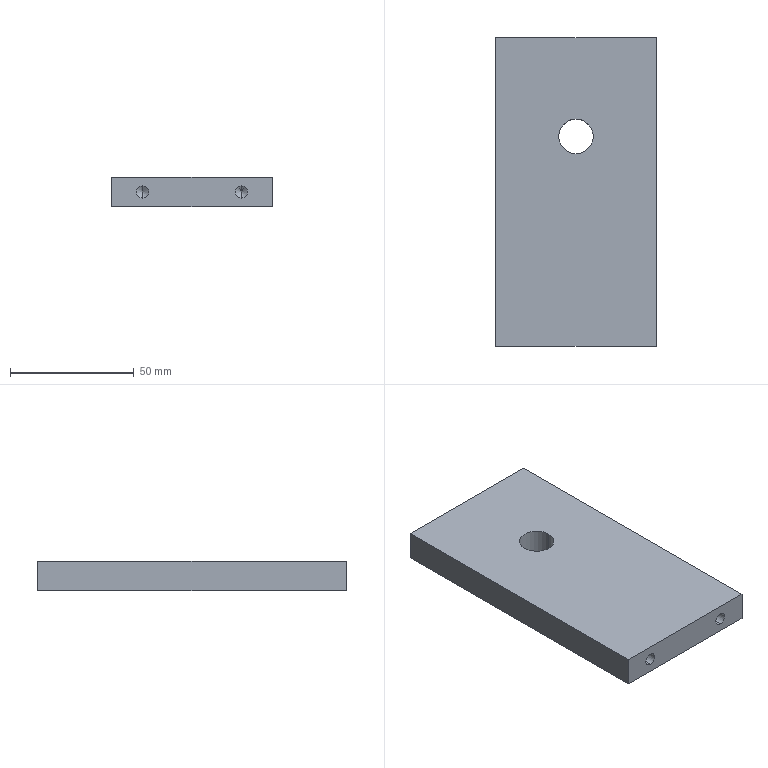Component | SolidWorks | TractionVerticalPlate-1 | 1 solid | 24 faces | box 65 x 125 x 12 mm | volume 94278 mm3 | cylinder 10 | cone 8 | plane 6 | commonest cylinder face diameters 5 x8 14 x2
build123d program:
from build123d import *

# Parameters (mm, degrees)
SKETCH1_W             = 65
SKETCH1_H             = 125
SKETCH1_R             = 7
EXTRUDE1_DEPTH        = 12
M6_TAPPED_HOLE1_D     = 5
M6_TAPPED_HOLE1_DEPTH = 17
M6_TAPPED_HOLE1_TIP   = 1.502
M6_TAPPED_HOLE2_D     = 5
M6_TAPPED_HOLE2_DEPTH = 17
M6_TAPPED_HOLE2_TIP   = 1.502


with BuildPart() as part:
    # Sketch1 → Extrude1 (new body)
    with BuildSketch(Plane.XY):
        Rectangle(SKETCH1_W, SKETCH1_H)
        with Locations((0, 22.5)):
            Circle(SKETCH1_R, mode=Mode.SUBTRACT)
    extrude(amount=EXTRUDE1_DEPTH)

    # M6 Tapped Hole1
    with Locations(Plane(origin=(0, 62.5, 0), x_dir=(-1, 0, 0), z_dir=(0, 1, 0))):
        with Locations((20, 6), (-20, 6)):
            Hole(M6_TAPPED_HOLE1_D / 2, depth=M6_TAPPED_HOLE1_DEPTH)
            with Locations((0, 0, -(M6_TAPPED_HOLE1_DEPTH + M6_TAPPED_HOLE1_TIP / 2))):  # 118° drill point
                Cone(0, M6_TAPPED_HOLE1_D / 2, M6_TAPPED_HOLE1_TIP, mode=Mode.SUBTRACT)

    # M6 Tapped Hole2
    with Locations(Plane.XZ.offset(62.5)):
        with Locations((20, 6), (-20, 6)):
            Hole(M6_TAPPED_HOLE2_D / 2, depth=M6_TAPPED_HOLE2_DEPTH)
            with Locations((0, 0, -(M6_TAPPED_HOLE2_DEPTH + M6_TAPPED_HOLE2_TIP / 2))):  # 118° drill point
                Cone(0, M6_TAPPED_HOLE2_D / 2, M6_TAPPED_HOLE2_TIP, mode=Mode.SUBTRACT)


solid = part.part

# Placed as in the assembly
solid = solid.moved(Location((250.216, 449.483, 260.5), (0, 0, 0)))
STEP:
#1=COLOUR_RGB('',0.7922,0.8196,0.9333);
#2=FILL_AREA_STYLE_COLOUR('',#1);
#3=FILL_AREA_STYLE('',(#2));
#4=SURFACE_STYLE_FILL_AREA(#3);
#5=SURFACE_SIDE_STYLE('',(#4));
#6=SURFACE_STYLE_USAGE(.BOTH.,#5);
#7=PRESENTATION_STYLE_ASSIGNMENT((#6));
#8=CARTESIAN_POINT('',(10.638,15.905,10.591));
#9=VERTEX_POINT('',#8);
#10=CARTESIAN_POINT('',(10.638,15.905,10.394));
#11=VERTEX_POINT('',#10);
#12=CARTESIAN_POINT('',(10.638,15.905,10.492));
#13=DIRECTION('',(0.,-1.,0.));
#14=DIRECTION('',(0.,0.,-1.));
#15=AXIS2_PLACEMENT_3D('',#12,#13,#14);
#16=CIRCLE('',#15,0.09843);
#17=EDGE_CURVE('',#9,#11,#16,.T.);
#18=ORIENTED_EDGE('',*,*,#17,.F.);
#19=CARTESIAN_POINT('',(10.638,15.236,10.591));
#20=VERTEX_POINT('',#19);
#21=CARTESIAN_POINT('',(10.638,15.236,10.591));
#22=DIRECTION('',(0.,-1.,0.));
#23=VECTOR('',#22,39.37);
#24=LINE('',#21,#23);
#25=EDGE_CURVE('',#9,#20,#24,.T.);
#26=ORIENTED_EDGE('',*,*,#25,.T.);
#27=CARTESIAN_POINT('',(10.638,15.236,10.394));
#28=VERTEX_POINT('',#27);
#29=CARTESIAN_POINT('',(10.638,15.236,10.492));
#30=DIRECTION('',(0.,-1.,0.));
#31=DIRECTION('',(0.,0.,-1.));
#32=AXIS2_PLACEMENT_3D('',#29,#30,#31);
#33=CIRCLE('',#32,0.09843);
#34=EDGE_CURVE('',#20,#28,#33,.T.);
#35=ORIENTED_EDGE('',*,*,#34,.T.);
#36=CARTESIAN_POINT('',(10.638,15.236,10.394));
#37=DIRECTION('',(0.,-1.,0.));
#38=VECTOR('',#37,39.37);
#39=LINE('',#36,#38);
#40=EDGE_CURVE('',#11,#28,#39,.T.);
#41=ORIENTED_EDGE('',*,*,#40,.F.);
#42=EDGE_LOOP('',(#18,#26,#35,#41));
#43=FACE_OUTER_BOUND('',#42,.T.);
#44=CARTESIAN_POINT('',(10.638,15.236,10.492));
#45=DIRECTION('',(0.,-1.,0.));
#46=DIRECTION('',(0.,0.,-1.));
#47=AXIS2_PLACEMENT_3D('',#44,#45,#46);
#48=CYLINDRICAL_SURFACE('',#47,0.09843);
#49=ADVANCED_FACE('',(#43),#48,.F.);
#50=CARTESIAN_POINT('',(10.638,15.964,10.492));
#51=VERTEX_POINT('',#50);
#52=CARTESIAN_POINT('',(10.638,15.905,10.394));
#53=DIRECTION('',(0.,-0.515,-0.8572));
#54=VECTOR('',#53,39.37);
#55=LINE('',#52,#54);
#56=EDGE_CURVE('',#51,#11,#55,.T.);
#57=ORIENTED_EDGE('',*,*,#56,.F.);
#58=CARTESIAN_POINT('',(10.638,15.905,10.591));
#59=DIRECTION('',(0.,-0.515,0.8572));
#60=VECTOR('',#59,39.37);
#61=LINE('',#58,#60);
#62=EDGE_CURVE('',#51,#9,#61,.T.);
#63=ORIENTED_EDGE('',*,*,#62,.T.);
#64=ORIENTED_EDGE('',*,*,#17,.T.);
#65=EDGE_LOOP('',(#57,#63,#64));
#66=FACE_OUTER_BOUND('',#65,.T.);
#67=CARTESIAN_POINT('',(10.638,15.905,10.492));
#68=DIRECTION('',(0.,-1.,0.));
#69=DIRECTION('',(0.,0.,-1.));
#70=AXIS2_PLACEMENT_3D('',#67,#68,#69);
#71=CONICAL_SURFACE('',#70,0.09843,1.03);
#72=ADVANCED_FACE('',(#66),#71,.F.);
#73=CARTESIAN_POINT('',(9.064,15.905,10.591));
#74=VERTEX_POINT('',#73);
#75=CARTESIAN_POINT('',(9.064,15.905,10.394));
#76=VERTEX_POINT('',#75);
#77=CARTESIAN_POINT('',(9.064,15.905,10.492));
#78=DIRECTION('',(0.,-1.,0.));
#79=DIRECTION('',(0.,0.,-1.));
#80=AXIS2_PLACEMENT_3D('',#77,#78,#79);
#81=CIRCLE('',#80,0.09843);
#82=EDGE_CURVE('',#74,#76,#81,.T.);
#83=ORIENTED_EDGE('',*,*,#82,.F.);
#84=CARTESIAN_POINT('',(9.064,15.236,10.591));
#85=VERTEX_POINT('',#84);
#86=CARTESIAN_POINT('',(9.064,15.236,10.591));
#87=DIRECTION('',(0.,-1.,0.));
#88=VECTOR('',#87,39.37);
#89=LINE('',#86,#88);
#90=EDGE_CURVE('',#74,#85,#89,.T.);
#91=ORIENTED_EDGE('',*,*,#90,.T.);
#92=CARTESIAN_POINT('',(9.064,15.236,10.394));
#93=VERTEX_POINT('',#92);
#94=CARTESIAN_POINT('',(9.064,15.236,10.492));
#95=DIRECTION('',(0.,-1.,0.));
#96=DIRECTION('',(0.,0.,-1.));
#97=AXIS2_PLACEMENT_3D('',#94,#95,#96);
#98=CIRCLE('',#97,0.09843);
#99=EDGE_CURVE('',#85,#93,#98,.T.);
#100=ORIENTED_EDGE('',*,*,#99,.T.);
#101=CARTESIAN_POINT('',(9.064,15.236,10.394));
#102=DIRECTION('',(0.,-1.,0.));
#103=VECTOR('',#102,39.37);
#104=LINE('',#101,#103);
#105=EDGE_CURVE('',#76,#93,#104,.T.);
#106=ORIENTED_EDGE('',*,*,#105,.F.);
#107=EDGE_LOOP('',(#83,#91,#100,#106));
#108=FACE_OUTER_BOUND('',#107,.T.);
#109=CARTESIAN_POINT('',(9.064,15.236,10.492));
#110=DIRECTION('',(0.,-1.,0.));
#111=DIRECTION('',(0.,0.,-1.));
#112=AXIS2_PLACEMENT_3D('',#109,#110,#111);
#113=CYLINDRICAL_SURFACE('',#112,0.09843);
#114=ADVANCED_FACE('',(#108),#113,.F.);
#115=CARTESIAN_POINT('',(9.064,15.964,10.492));
#116=VERTEX_POINT('',#115);
#117=CARTESIAN_POINT('',(9.064,15.905,10.394));
#118=DIRECTION('',(0.,-0.515,-0.8572));
#119=VECTOR('',#118,39.37);
#120=LINE('',#117,#119);
#121=EDGE_CURVE('',#116,#76,#120,.T.);
#122=ORIENTED_EDGE('',*,*,#121,.F.);
#123=CARTESIAN_POINT('',(9.064,15.905,10.591));
#124=DIRECTION('',(0.,-0.515,0.8572));
#125=VECTOR('',#124,39.37);
#126=LINE('',#123,#125);
#127=EDGE_CURVE('',#116,#74,#126,.T.);
#128=ORIENTED_EDGE('',*,*,#127,.T.);
#129=ORIENTED_EDGE('',*,*,#82,.T.);
#130=EDGE_LOOP('',(#122,#128,#129));
#131=FACE_OUTER_BOUND('',#130,.T.);
#132=CARTESIAN_POINT('',(9.064,15.905,10.492));
#133=DIRECTION('',(0.,-1.,0.));
#134=DIRECTION('',(0.,0.,-1.));
#135=AXIS2_PLACEMENT_3D('',#132,#133,#134);
#136=CONICAL_SURFACE('',#135,0.09843,1.03);
#137=ADVANCED_FACE('',(#131),#136,.F.);
#138=CARTESIAN_POINT('',(9.064,19.488,10.394));
#139=VERTEX_POINT('',#138);
#140=CARTESIAN_POINT('',(9.064,19.488,10.591));
#141=VERTEX_POINT('',#140);
#142=CARTESIAN_POINT('',(9.064,19.488,10.492));
#143=DIRECTION('',(0.,1.,0.));
#144=DIRECTION('',(0.,0.,1.));
#145=AXIS2_PLACEMENT_3D('',#142,#143,#144);
#146=CIRCLE('',#145,0.09843);
#147=EDGE_CURVE('',#139,#141,#146,.T.);
#148=ORIENTED_EDGE('',*,*,#147,.F.);
#149=CARTESIAN_POINT('',(9.064,20.157,10.394));
#150=VERTEX_POINT('',#149);
#151=CARTESIAN_POINT('',(9.064,20.157,10.394));
#152=DIRECTION('',(0.,1.,0.));
#153=VECTOR('',#152,39.37);
#154=LINE('',#151,#153);
#155=EDGE_CURVE('',#139,#150,#154,.T.);
#156=ORIENTED_EDGE('',*,*,#155,.T.);
#157=CARTESIAN_POINT('',(9.064,20.157,10.591));
#158=VERTEX_POINT('',#157);
#159=CARTESIAN_POINT('',(9.064,20.157,10.492));
#160=DIRECTION('',(0.,1.,0.));
#161=DIRECTION('',(0.,0.,1.));
#162=AXIS2_PLACEMENT_3D('',#159,#160,#161);
#163=CIRCLE('',#162,0.09843);
#164=EDGE_CURVE('',#150,#158,#163,.T.);
#165=ORIENTED_EDGE('',*,*,#164,.T.);
#166=CARTESIAN_POINT('',(9.064,20.157,10.591));
#167=DIRECTION('',(0.,1.,0.));
#168=VECTOR('',#167,39.37);
#169=LINE('',#166,#168);
#170=EDGE_CURVE('',#141,#158,#169,.T.);
#171=ORIENTED_EDGE('',*,*,#170,.F.);
#172=EDGE_LOOP('',(#148,#156,#165,#171));
#173=FACE_OUTER_BOUND('',#172,.T.);
#174=CARTESIAN_POINT('',(9.064,20.157,10.492));
#175=DIRECTION('',(0.,1.,0.));
#176=DIRECTION('',(0.,0.,1.));
#177=AXIS2_PLACEMENT_3D('',#174,#175,#176);
#178=CYLINDRICAL_SURFACE('',#177,0.09843);
#179=ADVANCED_FACE('',(#173),#178,.F.);
#180=CARTESIAN_POINT('',(9.064,19.428,10.492));
#181=VERTEX_POINT('',#180);
#182=CARTESIAN_POINT('',(9.064,19.488,10.591));
#183=DIRECTION('',(0.,0.515,0.8572));
#184=VECTOR('',#183,39.37);
#185=LINE('',#182,#184);
#186=EDGE_CURVE('',#181,#141,#185,.T.);
#187=ORIENTED_EDGE('',*,*,#186,.F.);
#188=CARTESIAN_POINT('',(9.064,19.488,10.394));
#189=DIRECTION('',(0.,0.515,-0.8572));
#190=VECTOR('',#189,39.37);
#191=LINE('',#188,#190);
#192=EDGE_CURVE('',#181,#139,#191,.T.);
#193=ORIENTED_EDGE('',*,*,#192,.T.);
#194=ORIENTED_EDGE('',*,*,#147,.T.);
#195=EDGE_LOOP('',(#187,#193,#194));
#196=FACE_OUTER_BOUND('',#195,.T.);
#197=CARTESIAN_POINT('',(9.064,19.488,10.492));
#198=DIRECTION('',(0.,1.,0.));
#199=DIRECTION('',(0.,0.,1.));
#200=AXIS2_PLACEMENT_3D('',#197,#198,#199);
#201=CONICAL_SURFACE('',#200,0.09843,1.03);
#202=ADVANCED_FACE('',(#196),#201,.F.);
#203=CARTESIAN_POINT('',(10.638,19.488,10.394));
#204=VERTEX_POINT('',#203);
#205=CARTESIAN_POINT('',(10.638,19.488,10.591));
#206=VERTEX_POINT('',#205);
#207=CARTESIAN_POINT('',(10.638,19.488,10.492));
#208=DIRECTION('',(0.,1.,0.));
#209=DIRECTION('',(0.,0.,1.));
#210=AXIS2_PLACEMENT_3D('',#207,#208,#209);
#211=CIRCLE('',#210,0.09843);
#212=EDGE_CURVE('',#204,#206,#211,.T.);
#213=ORIENTED_EDGE('',*,*,#212,.F.);
#214=CARTESIAN_POINT('',(10.638,20.157,10.394));
#215=VERTEX_POINT('',#214);
#216=CARTESIAN_POINT('',(10.638,20.157,10.394));
#217=DIRECTION('',(0.,1.,0.));
#218=VECTOR('',#217,39.37);
#219=LINE('',#216,#218);
#220=EDGE_CURVE('',#204,#215,#219,.T.);
#221=ORIENTED_EDGE('',*,*,#220,.T.);
#222=CARTESIAN_POINT('',(10.638,20.157,10.591));
#223=VERTEX_POINT('',#222);
#224=CARTESIAN_POINT('',(10.638,20.157,10.492));
#225=DIRECTION('',(0.,1.,0.));
#226=DIRECTION('',(0.,0.,1.));
#227=AXIS2_PLACEMENT_3D('',#224,#225,#226);
#228=CIRCLE('',#227,0.09843);
#229=EDGE_CURVE('',#215,#223,#228,.T.);
#230=ORIENTED_EDGE('',*,*,#229,.T.);
#231=CARTESIAN_POINT('',(10.638,20.157,10.591));
#232=DIRECTION('',(0.,1.,0.));
#233=VECTOR('',#232,39.37);
#234=LINE('',#231,#233);
#235=EDGE_CURVE('',#206,#223,#234,.T.);
#236=ORIENTED_EDGE('',*,*,#235,.F.);
#237=EDGE_LOOP('',(#213,#221,#230,#236));
#238=FACE_OUTER_BOUND('',#237,.T.);
#239=CARTESIAN_POINT('',(10.638,20.157,10.492));
#240=DIRECTION('',(0.,1.,0.));
#241=DIRECTION('',(0.,0.,1.));
#242=AXIS2_PLACEMENT_3D('',#239,#240,#241);
#243=CYLINDRICAL_SURFACE('',#242,0.09843);
#244=ADVANCED_FACE('',(#238),#243,.F.);
#245=CARTESIAN_POINT('',(10.638,19.428,10.492));
#246=VERTEX_POINT('',#245);
#247=CARTESIAN_POINT('',(10.638,19.488,10.591));
#248=DIRECTION('',(0.,0.515,0.8572));
#249=VECTOR('',#248,39.37);
#250=LINE('',#247,#249);
#251=EDGE_CURVE('',#246,#206,#250,.T.);
#252=ORIENTED_EDGE('',*,*,#251,.F.);
#253=CARTESIAN_POINT('',(10.638,19.488,10.394));
#254=DIRECTION('',(0.,0.515,-0.8572));
#255=VECTOR('',#254,39.37);
#256=LINE('',#253,#255);
#257=EDGE_CURVE('',#246,#204,#256,.T.);
#258=ORIENTED_EDGE('',*,*,#257,.T.);
#259=ORIENTED_EDGE('',*,*,#212,.T.);
#260=EDGE_LOOP('',(#252,#258,#259));
#261=FACE_OUTER_BOUND('',#260,.T.);
#262=CARTESIAN_POINT('',(10.638,19.488,10.492));
#263=DIRECTION('',(0.,1.,0.));
#264=DIRECTION('',(0.,0.,1.));
#265=AXIS2_PLACEMENT_3D('',#262,#263,#264);
#266=CONICAL_SURFACE('',#265,0.09843,1.03);
#267=ADVANCED_FACE('',(#261),#266,.F.);
#268=CARTESIAN_POINT('',(9.575,18.582,10.728));
#269=VERTEX_POINT('',#268);
#270=CARTESIAN_POINT('',(10.127,18.582,10.728));
#271=VERTEX_POINT('',#270);
#272=CARTESIAN_POINT('',(9.851,18.582,10.728));
#273=DIRECTION('',(0.,0.,1.));
#274=DIRECTION('',(1.,0.,0.));
#275=AXIS2_PLACEMENT_3D('',#272,#273,#274);
#276=CIRCLE('',#275,0.2756);
#277=EDGE_CURVE('',#269,#271,#276,.T.);
#278=ORIENTED_EDGE('',*,*,#277,.T.);
#279=CARTESIAN_POINT('',(10.127,18.582,10.256));
#280=VERTEX_POINT('',#279);
#281=CARTESIAN_POINT('',(10.127,18.582,10.728));
#282=DIRECTION('',(0.,0.,-1.));
#283=VECTOR('',#282,39.37);
#284=LINE('',#281,#283);
#285=EDGE_CURVE('',#271,#280,#284,.T.);
#286=ORIENTED_EDGE('',*,*,#285,.T.);
#287=CARTESIAN_POINT('',(9.575,18.582,10.256));
#288=VERTEX_POINT('',#287);
#289=CARTESIAN_POINT('',(9.851,18.582,10.256));
#290=DIRECTION('',(0.,0.,1.));
#291=DIRECTION('',(1.,0.,0.));
#292=AXIS2_PLACEMENT_3D('',#289,#290,#291);
#293=CIRCLE('',#292,0.2756);
#294=EDGE_CURVE('',#288,#280,#293,.T.);
#295=ORIENTED_EDGE('',*,*,#294,.F.);
#296=CARTESIAN_POINT('',(9.575,18.582,10.728));
#297=DIRECTION('',(0.,0.,-1.));
#298=VECTOR('',#297,39.37);
#299=LINE('',#296,#298);
#300=EDGE_CURVE('',#269,#288,#299,.T.);
#301=ORIENTED_EDGE('',*,*,#300,.F.);
#302=EDGE_LOOP('',(#278,#286,#295,#301));
#303=FACE_OUTER_BOUND('',#302,.T.);
#304=CARTESIAN_POINT('',(9.851,18.582,10.728));
#305=DIRECTION('',(0.,0.,-1.));
#306=DIRECTION('',(-1.,0.,0.));
#307=AXIS2_PLACEMENT_3D('',#304,#305,#306);
#308=CYLINDRICAL_SURFACE('',#307,0.2756);
#309=ADVANCED_FACE('',(#303),#308,.F.);
#310=CARTESIAN_POINT('',(8.572,20.157,10.728));
#311=VERTEX_POINT('',#310);
#312=CARTESIAN_POINT('',(8.572,15.236,10.728));
#313=VERTEX_POINT('',#312);
#314=CARTESIAN_POINT('',(8.572,20.157,10.728));
#315=DIRECTION('',(0.,-1.,0.));
#316=VECTOR('',#315,39.37);
#317=LINE('',#314,#316);
#318=EDGE_CURVE('',#311,#313,#317,.T.);
#319=ORIENTED_EDGE('',*,*,#318,.T.);
#320=CARTESIAN_POINT('',(11.131,15.236,10.728));
#321=VERTEX_POINT('',#320);
#322=CARTESIAN_POINT('',(8.572,15.236,10.728));
#323=DIRECTION('',(1.,0.,0.));
#324=VECTOR('',#323,39.37);
#325=LINE('',#322,#324);
#326=EDGE_CURVE('',#313,#321,#325,.T.);
#327=ORIENTED_EDGE('',*,*,#326,.T.);
#328=CARTESIAN_POINT('',(11.131,20.157,10.728));
#329=VERTEX_POINT('',#328);
#330=CARTESIAN_POINT('',(11.131,20.157,10.728));
#331=DIRECTION('',(0.,1.,0.));
#332=VECTOR('',#331,39.37);
#333=LINE('',#330,#332);
#334=EDGE_CURVE('',#321,#329,#333,.T.);
#335=ORIENTED_EDGE('',*,*,#334,.T.);
#336=CARTESIAN_POINT('',(8.572,20.157,10.728));
#337=DIRECTION('',(-1.,0.,0.));
#338=VECTOR('',#337,39.37);
#339=LINE('',#336,#338);
#340=EDGE_CURVE('',#329,#311,#339,.T.);
#341=ORIENTED_EDGE('',*,*,#340,.T.);
#342=EDGE_LOOP('',(#319,#327,#335,#341));
#343=FACE_OUTER_BOUND('',#342,.T.);
#344=ORIENTED_EDGE('',*,*,#277,.F.);
#345=CARTESIAN_POINT('',(9.851,18.582,10.728));
#346=DIRECTION('',(0.,0.,1.));
#347=DIRECTION('',(1.,0.,0.));
#348=AXIS2_PLACEMENT_3D('',#345,#346,#347);
#349=CIRCLE('',#348,0.2756);
#350=EDGE_CURVE('',#271,#269,#349,.T.);
#351=ORIENTED_EDGE('',*,*,#350,.F.);
#352=EDGE_LOOP('',(#344,#351));
#353=FACE_BOUND('',#352,.T.);
#354=CARTESIAN_POINT('',(8.572,15.236,10.728));
#355=DIRECTION('',(0.,0.,1.));
#356=DIRECTION('',(1.,0.,0.));
#357=AXIS2_PLACEMENT_3D('',#354,#355,#356);
#358=PLANE('',#357);
#359=ADVANCED_FACE('',(#343,#353),#358,.T.);
#360=CARTESIAN_POINT('',(8.572,20.157,10.256));
#361=VERTEX_POINT('',#360);
#362=CARTESIAN_POINT('',(8.572,15.236,10.256));
#363=VERTEX_POINT('',#362);
#364=CARTESIAN_POINT('',(8.572,20.157,10.256));
#365=DIRECTION('',(0.,-1.,0.));
#366=VECTOR('',#365,39.37);
#367=LINE('',#364,#366);
#368=EDGE_CURVE('',#361,#363,#367,.T.);
#369=ORIENTED_EDGE('',*,*,#368,.F.);
#370=CARTESIAN_POINT('',(11.131,20.157,10.256));
#371=VERTEX_POINT('',#370);
#372=CARTESIAN_POINT('',(8.572,20.157,10.256));
#373=DIRECTION('',(-1.,0.,0.));
#374=VECTOR('',#373,39.37);
#375=LINE('',#372,#374);
#376=EDGE_CURVE('',#371,#361,#375,.T.);
#377=ORIENTED_EDGE('',*,*,#376,.F.);
#378=CARTESIAN_POINT('',(11.131,15.236,10.256));
#379=VERTEX_POINT('',#378);
#380=CARTESIAN_POINT('',(11.131,20.157,10.256));
#381=DIRECTION('',(0.,1.,0.));
#382=VECTOR('',#381,39.37);
#383=LINE('',#380,#382);
#384=EDGE_CURVE('',#379,#371,#383,.T.);
#385=ORIENTED_EDGE('',*,*,#384,.F.);
#386=CARTESIAN_POINT('',(8.572,15.236,10.256));
#387=DIRECTION('',(1.,0.,0.));
#388=VECTOR('',#387,39.37);
#389=LINE('',#386,#388);
#390=EDGE_CURVE('',#363,#379,#389,.T.);
#391=ORIENTED_EDGE('',*,*,#390,.F.);
#392=EDGE_LOOP('',(#369,#377,#385,#391));
#393=FACE_OUTER_BOUND('',#392,.T.);
#394=ORIENTED_EDGE('',*,*,#294,.T.);
#395=CARTESIAN_POINT('',(9.851,18.582,10.256));
#396=DIRECTION('',(0.,0.,1.));
#397=DIRECTION('',(1.,0.,0.));
#398=AXIS2_PLACEMENT_3D('',#395,#396,#397);
#399=CIRCLE('',#398,0.2756);
#400=EDGE_CURVE('',#280,#288,#399,.T.);
#401=ORIENTED_EDGE('',*,*,#400,.T.);
#402=EDGE_LOOP('',(#394,#401));
#403=FACE_BOUND('',#402,.T.);
#404=CARTESIAN_POINT('',(8.572,15.236,10.256));
#405=DIRECTION('',(0.,0.,1.));
#406=DIRECTION('',(1.,0.,0.));
#407=AXIS2_PLACEMENT_3D('',#404,#405,#406);
#408=PLANE('',#407);
#409=ADVANCED_FACE('',(#393,#403),#408,.F.);
#410=ORIENTED_EDGE('',*,*,#368,.T.);
#411=CARTESIAN_POINT('',(8.572,15.236,10.728));
#412=DIRECTION('',(0.,0.,-1.));
#413=VECTOR('',#412,39.37);
#414=LINE('',#411,#413);
#415=EDGE_CURVE('',#313,#363,#414,.T.);
#416=ORIENTED_EDGE('',*,*,#415,.F.);
#417=ORIENTED_EDGE('',*,*,#318,.F.);
#418=CARTESIAN_POINT('',(8.572,20.157,10.728));
#419=DIRECTION('',(0.,0.,-1.));
#420=VECTOR('',#419,39.37);
#421=LINE('',#418,#420);
#422=EDGE_CURVE('',#311,#361,#421,.T.);
#423=ORIENTED_EDGE('',*,*,#422,.T.);
#424=EDGE_LOOP('',(#410,#416,#417,#423));
#425=FACE_OUTER_BOUND('',#424,.T.);
#426=CARTESIAN_POINT('',(8.572,20.157,10.728));
#427=DIRECTION('',(1.,0.,0.));
#428=DIRECTION('',(0.,0.,-1.));
#429=AXIS2_PLACEMENT_3D('',#426,#427,#428);
#430=PLANE('',#429);
#431=ADVANCED_FACE('',(#425),#430,.F.);
#432=CARTESIAN_POINT('',(10.638,15.236,10.492));
#433=DIRECTION('',(0.,-1.,0.));
#434=DIRECTION('',(0.,0.,-1.));
#435=AXIS2_PLACEMENT_3D('',#432,#433,#434);
#436=CIRCLE('',#435,0.09843);
#437=EDGE_CURVE('',#28,#20,#436,.T.);
#438=ORIENTED_EDGE('',*,*,#437,.F.);
#439=ORIENTED_EDGE('',*,*,#34,.F.);
#440=EDGE_LOOP('',(#438,#439));
#441=FACE_BOUND('',#440,.T.);
#442=CARTESIAN_POINT('',(9.064,15.236,10.492));
#443=DIRECTION('',(0.,-1.,0.));
#444=DIRECTION('',(0.,0.,-1.));
#445=AXIS2_PLACEMENT_3D('',#442,#443,#444);
#446=CIRCLE('',#445,0.09843);
#447=EDGE_CURVE('',#93,#85,#446,.T.);
#448=ORIENTED_EDGE('',*,*,#447,.F.);
#449=ORIENTED_EDGE('',*,*,#99,.F.);
#450=EDGE_LOOP('',(#448,#449));
#451=FACE_BOUND('',#450,.T.);
#452=ORIENTED_EDGE('',*,*,#390,.T.);
#453=CARTESIAN_POINT('',(11.131,15.236,10.728));
#454=DIRECTION('',(0.,0.,-1.));
#455=VECTOR('',#454,39.37);
#456=LINE('',#453,#455);
#457=EDGE_CURVE('',#321,#379,#456,.T.);
#458=ORIENTED_EDGE('',*,*,#457,.F.);
#459=ORIENTED_EDGE('',*,*,#326,.F.);
#460=ORIENTED_EDGE('',*,*,#415,.T.);
#461=EDGE_LOOP('',(#452,#458,#459,#460));
#462=FACE_OUTER_BOUND('',#461,.T.);
#463=CARTESIAN_POINT('',(8.572,15.236,10.728));
#464=DIRECTION('',(0.,1.,0.));
#465=DIRECTION('',(0.,0.,1.));
#466=AXIS2_PLACEMENT_3D('',#463,#464,#465);
#467=PLANE('',#466);
#468=ADVANCED_FACE('',(#441,#451,#462),#467,.F.);
#469=ORIENTED_EDGE('',*,*,#384,.T.);
#470=CARTESIAN_POINT('',(11.131,20.157,10.728));
#471=DIRECTION('',(0.,0.,-1.));
#472=VECTOR('',#471,39.37);
#473=LINE('',#470,#472);
#474=EDGE_CURVE('',#329,#371,#473,.T.);
#475=ORIENTED_EDGE('',*,*,#474,.F.);
#476=ORIENTED_EDGE('',*,*,#334,.F.);
#477=ORIENTED_EDGE('',*,*,#457,.T.);
#478=EDGE_LOOP('',(#469,#475,#476,#477));
#479=FACE_OUTER_BOUND('',#478,.T.);
#480=CARTESIAN_POINT('',(11.131,20.157,10.728));
#481=DIRECTION('',(-1.,0.,0.));
#482=DIRECTION('',(0.,0.,1.));
#483=AXIS2_PLACEMENT_3D('',#480,#481,#482);
#484=PLANE('',#483);
#485=ADVANCED_FACE('',(#479),#484,.F.);
#486=CARTESIAN_POINT('',(9.064,20.157,10.492));
#487=DIRECTION('',(0.,1.,0.));
#488=DIRECTION('',(0.,0.,1.));
#489=AXIS2_PLACEMENT_3D('',#486,#487,#488);
#490=CIRCLE('',#489,0.09843);
#491=EDGE_CURVE('',#158,#150,#490,.T.);
#492=ORIENTED_EDGE('',*,*,#491,.F.);
#493=ORIENTED_EDGE('',*,*,#164,.F.);
#494=EDGE_LOOP('',(#492,#493));
#495=FACE_BOUND('',#494,.T.);
#496=CARTESIAN_POINT('',(10.638,20.157,10.492));
#497=DIRECTION('',(0.,1.,0.));
#498=DIRECTION('',(0.,0.,1.));
#499=AXIS2_PLACEMENT_3D('',#496,#497,#498);
#500=CIRCLE('',#499,0.09843);
#501=EDGE_CURVE('',#223,#215,#500,.T.);
#502=ORIENTED_EDGE('',*,*,#501,.F.);
#503=ORIENTED_EDGE('',*,*,#229,.F.);
#504=EDGE_LOOP('',(#502,#503));
#505=FACE_BOUND('',#504,.T.);
#506=ORIENTED_EDGE('',*,*,#376,.T.);
#507=ORIENTED_EDGE('',*,*,#422,.F.);
#508=ORIENTED_EDGE('',*,*,#340,.F.);
#509=ORIENTED_EDGE('',*,*,#474,.T.);
#510=EDGE_LOOP('',(#506,#507,#508,#509));
#511=FACE_OUTER_BOUND('',#510,.T.);
#512=CARTESIAN_POINT('',(8.572,20.157,10.728));
#513=DIRECTION('',(0.,-1.,0.));
#514=DIRECTION('',(0.,0.,-1.));
#515=AXIS2_PLACEMENT_3D('',#512,#513,#514);
#516=PLANE('',#515);
#517=ADVANCED_FACE('',(#495,#505,#511),#516,.F.);
#518=ORIENTED_EDGE('',*,*,#285,.F.);
#519=ORIENTED_EDGE('',*,*,#350,.T.);
#520=ORIENTED_EDGE('',*,*,#300,.T.);
#521=ORIENTED_EDGE('',*,*,#400,.F.);
#522=EDGE_LOOP('',(#518,#519,#520,#521));
#523=FACE_OUTER_BOUND('',#522,.T.);
#524=CARTESIAN_POINT('',(9.851,18.582,10.728));
#525=DIRECTION('',(0.,0.,-1.));
#526=DIRECTION('',(-1.,0.,0.));
#527=AXIS2_PLACEMENT_3D('',#524,#525,#526);
#528=CYLINDRICAL_SURFACE('',#527,0.2756);
#529=ADVANCED_FACE('',(#523),#528,.F.);
#530=ORIENTED_EDGE('',*,*,#257,.F.);
#531=ORIENTED_EDGE('',*,*,#251,.T.);
#532=CARTESIAN_POINT('',(10.638,19.488,10.492));
#533=DIRECTION('',(0.,1.,0.));
#534=DIRECTION('',(0.,0.,1.));
#535=AXIS2_PLACEMENT_3D('',#532,#533,#534);
#536=CIRCLE('',#535,0.09843);
#537=EDGE_CURVE('',#206,#204,#536,.T.);
#538=ORIENTED_EDGE('',*,*,#537,.T.);
#539=EDGE_LOOP('',(#530,#531,#538));
#540=FACE_OUTER_BOUND('',#539,.T.);
#541=CARTESIAN_POINT('',(10.638,19.488,10.492));
#542=DIRECTION('',(0.,1.,0.));
#543=DIRECTION('',(0.,0.,1.));
#544=AXIS2_PLACEMENT_3D('',#541,#542,#543);
#545=CONICAL_SURFACE('',#544,0.09843,1.03);
#546=ADVANCED_FACE('',(#540),#545,.F.);
#547=ORIENTED_EDGE('',*,*,#220,.F.);
#548=ORIENTED_EDGE('',*,*,#537,.F.);
#549=ORIENTED_EDGE('',*,*,#235,.T.);
#550=ORIENTED_EDGE('',*,*,#501,.T.);
#551=EDGE_LOOP('',(#547,#548,#549,#550));
#552=FACE_OUTER_BOUND('',#551,.T.);
#553=CARTESIAN_POINT('',(10.638,20.157,10.492));
#554=DIRECTION('',(0.,1.,0.));
#555=DIRECTION('',(0.,0.,1.));
#556=AXIS2_PLACEMENT_3D('',#553,#554,#555);
#557=CYLINDRICAL_SURFACE('',#556,0.09843);
#558=ADVANCED_FACE('',(#552),#557,.F.);
#559=ORIENTED_EDGE('',*,*,#192,.F.);
#560=ORIENTED_EDGE('',*,*,#186,.T.);
#561=CARTESIAN_POINT('',(9.064,19.488,10.492));
#562=DIRECTION('',(0.,1.,0.));
#563=DIRECTION('',(0.,0.,1.));
#564=AXIS2_PLACEMENT_3D('',#561,#562,#563);
#565=CIRCLE('',#564,0.09843);
#566=EDGE_CURVE('',#141,#139,#565,.T.);
#567=ORIENTED_EDGE('',*,*,#566,.T.);
#568=EDGE_LOOP('',(#559,#560,#567));
#569=FACE_OUTER_BOUND('',#568,.T.);
#570=CARTESIAN_POINT('',(9.064,19.488,10.492));
#571=DIRECTION('',(0.,1.,0.));
#572=DIRECTION('',(0.,0.,1.));
#573=AXIS2_PLACEMENT_3D('',#570,#571,#572);
#574=CONICAL_SURFACE('',#573,0.09843,1.03);
#575=ADVANCED_FACE('',(#569),#574,.F.);
#576=ORIENTED_EDGE('',*,*,#155,.F.);
#577=ORIENTED_EDGE('',*,*,#566,.F.);
#578=ORIENTED_EDGE('',*,*,#170,.T.);
#579=ORIENTED_EDGE('',*,*,#491,.T.);
#580=EDGE_LOOP('',(#576,#577,#578,#579));
#581=FACE_OUTER_BOUND('',#580,.T.);
#582=CARTESIAN_POINT('',(9.064,20.157,10.492));
#583=DIRECTION('',(0.,1.,0.));
#584=DIRECTION('',(0.,0.,1.));
#585=AXIS2_PLACEMENT_3D('',#582,#583,#584);
#586=CYLINDRICAL_SURFACE('',#585,0.09843);
#587=ADVANCED_FACE('',(#581),#586,.F.);
#588=ORIENTED_EDGE('',*,*,#127,.F.);
#589=ORIENTED_EDGE('',*,*,#121,.T.);
#590=CARTESIAN_POINT('',(9.064,15.905,10.492));
#591=DIRECTION('',(0.,-1.,0.));
#592=DIRECTION('',(0.,0.,-1.));
#593=AXIS2_PLACEMENT_3D('',#590,#591,#592);
#594=CIRCLE('',#593,0.09843);
#595=EDGE_CURVE('',#76,#74,#594,.T.);
#596=ORIENTED_EDGE('',*,*,#595,.T.);
#597=EDGE_LOOP('',(#588,#589,#596));
#598=FACE_OUTER_BOUND('',#597,.T.);
#599=CARTESIAN_POINT('',(9.064,15.905,10.492));
#600=DIRECTION('',(0.,-1.,0.));
#601=DIRECTION('',(0.,0.,-1.));
#602=AXIS2_PLACEMENT_3D('',#599,#600,#601);
#603=CONICAL_SURFACE('',#602,0.09843,1.03);
#604=ADVANCED_FACE('',(#598),#603,.F.);
#605=ORIENTED_EDGE('',*,*,#90,.F.);
#606=ORIENTED_EDGE('',*,*,#595,.F.);
#607=ORIENTED_EDGE('',*,*,#105,.T.);
#608=ORIENTED_EDGE('',*,*,#447,.T.);
#609=EDGE_LOOP('',(#605,#606,#607,#608));
#610=FACE_OUTER_BOUND('',#609,.T.);
#611=CARTESIAN_POINT('',(9.064,15.236,10.492));
#612=DIRECTION('',(0.,-1.,0.));
#613=DIRECTION('',(0.,0.,-1.));
#614=AXIS2_PLACEMENT_3D('',#611,#612,#613);
#615=CYLINDRICAL_SURFACE('',#614,0.09843);
#616=ADVANCED_FACE('',(#610),#615,.F.);
#617=ORIENTED_EDGE('',*,*,#62,.F.);
#618=ORIENTED_EDGE('',*,*,#56,.T.);
#619=CARTESIAN_POINT('',(10.638,15.905,10.492));
#620=DIRECTION('',(0.,-1.,0.));
#621=DIRECTION('',(0.,0.,-1.));
#622=AXIS2_PLACEMENT_3D('',#619,#620,#621);
#623=CIRCLE('',#622,0.09843);
#624=EDGE_CURVE('',#11,#9,#623,.T.);
#625=ORIENTED_EDGE('',*,*,#624,.T.);
#626=EDGE_LOOP('',(#617,#618,#625));
#627=FACE_OUTER_BOUND('',#626,.T.);
#628=CARTESIAN_POINT('',(10.638,15.905,10.492));
#629=DIRECTION('',(0.,-1.,0.));
#630=DIRECTION('',(0.,0.,-1.));
#631=AXIS2_PLACEMENT_3D('',#628,#629,#630);
#632=CONICAL_SURFACE('',#631,0.09843,1.03);
#633=ADVANCED_FACE('',(#627),#632,.F.);
#634=ORIENTED_EDGE('',*,*,#25,.F.);
#635=ORIENTED_EDGE('',*,*,#624,.F.);
#636=ORIENTED_EDGE('',*,*,#40,.T.);
#637=ORIENTED_EDGE('',*,*,#437,.T.);
#638=EDGE_LOOP('',(#634,#635,#636,#637));
#639=FACE_OUTER_BOUND('',#638,.T.);
#640=CARTESIAN_POINT('',(10.638,15.236,10.492));
#641=DIRECTION('',(0.,-1.,0.));
#642=DIRECTION('',(0.,0.,-1.));
#643=AXIS2_PLACEMENT_3D('',#640,#641,#642);
#644=CYLINDRICAL_SURFACE('',#643,0.09843);
#645=ADVANCED_FACE('',(#639),#644,.F.);
#646=CLOSED_SHELL('',(#49,#72,#114,#137,#179,#202,#244,#267,#309,#359,#409,#431,#468,#485,#517,#529,#546,#558,#575,#587,#604,#616,#633,#645));
#647=MANIFOLD_SOLID_BREP('',#646);
#648=STYLED_ITEM('',(#7),#647);
#649=PRESENTATION_LAYER_ASSIGNMENT('','',(#648));
#650=CARTESIAN_POINT('',(0.,0.,0.));
#651=DIRECTION('',(0.,0.,1.));
#652=DIRECTION('',(1.,0.,0.));
#653=AXIS2_PLACEMENT_3D('',#650,#651,#652);
#654=(LENGTH_UNIT()NAMED_UNIT(*)SI_UNIT($,.METRE.));
#655=LENGTH_MEASURE_WITH_UNIT(LENGTH_MEASURE(0.0254),#654);
#656=DIMENSIONAL_EXPONENTS(1.,0.,0.,0.,0.,0.,0.);
#657=(CONVERSION_BASED_UNIT('',#655)LENGTH_UNIT()NAMED_UNIT(#656));
#658=UNCERTAINTY_MEASURE_WITH_UNIT(LENGTH_MEASURE(0.00001),#657,'','');
#659=(NAMED_UNIT(*)PLANE_ANGLE_UNIT()SI_UNIT($,.RADIAN.));
#660=(NAMED_UNIT(*)SI_UNIT($,.STERADIAN.)SOLID_ANGLE_UNIT());
#661=(GEOMETRIC_REPRESENTATION_CONTEXT(3)GLOBAL_UNCERTAINTY_ASSIGNED_CONTEXT((#658))GLOBAL_UNIT_ASSIGNED_CONTEXT((#657,#659,#660))REPRESENTATION_CONTEXT('',''));
#662=ADVANCED_BREP_SHAPE_REPRESENTATION('',(#647,#653),#661);
#663=(LENGTH_UNIT()NAMED_UNIT(*)SI_UNIT($,.METRE.));
#664=LENGTH_MEASURE_WITH_UNIT(LENGTH_MEASURE(0.0254),#663);
#665=DIMENSIONAL_EXPONENTS(1.,0.,0.,0.,0.,0.,0.);
#666=(CONVERSION_BASED_UNIT('',#664)LENGTH_UNIT()NAMED_UNIT(#665));
#667=UNCERTAINTY_MEASURE_WITH_UNIT(LENGTH_MEASURE(0.00001),#666,'','');
#668=(NAMED_UNIT(*)PLANE_ANGLE_UNIT()SI_UNIT($,.RADIAN.));
#669=(NAMED_UNIT(*)SI_UNIT($,.STERADIAN.)SOLID_ANGLE_UNIT());
#670=(GEOMETRIC_REPRESENTATION_CONTEXT(3)GLOBAL_UNCERTAINTY_ASSIGNED_CONTEXT((#667))GLOBAL_UNIT_ASSIGNED_CONTEXT((#666,#668,#669))REPRESENTATION_CONTEXT('',''));
#671=MECHANICAL_DESIGN_GEOMETRIC_PRESENTATION_REPRESENTATION('',(#648),#670);